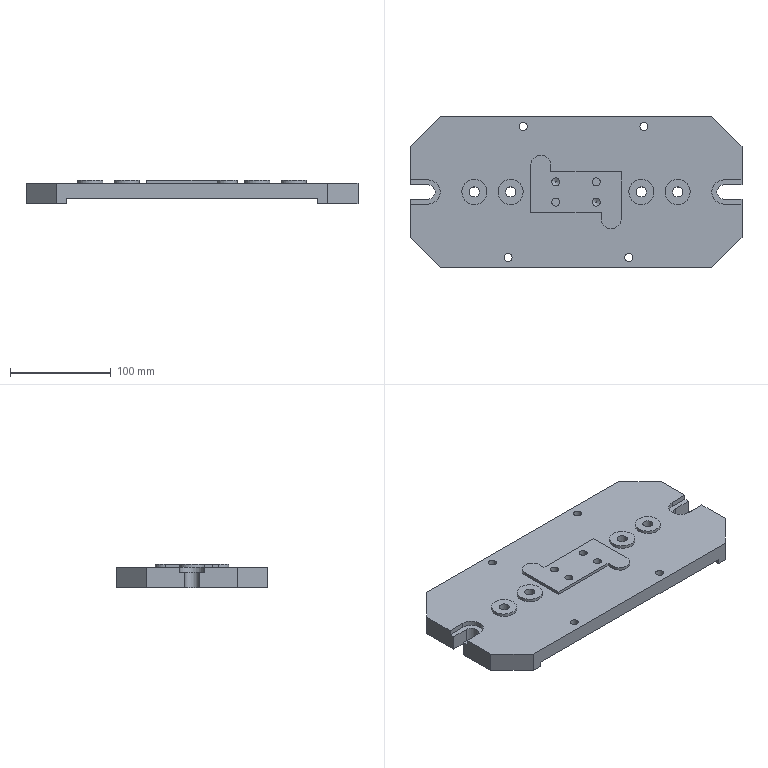Component | NX | JIG_BODY | 1 solid | 63 faces | volume 757097 mm3 | plane 39 | cylinder 22 | cone 2 | commonest cylinder face diameters 8 x8 25 x4 10 x4 20 x2 14 x2 24 x2